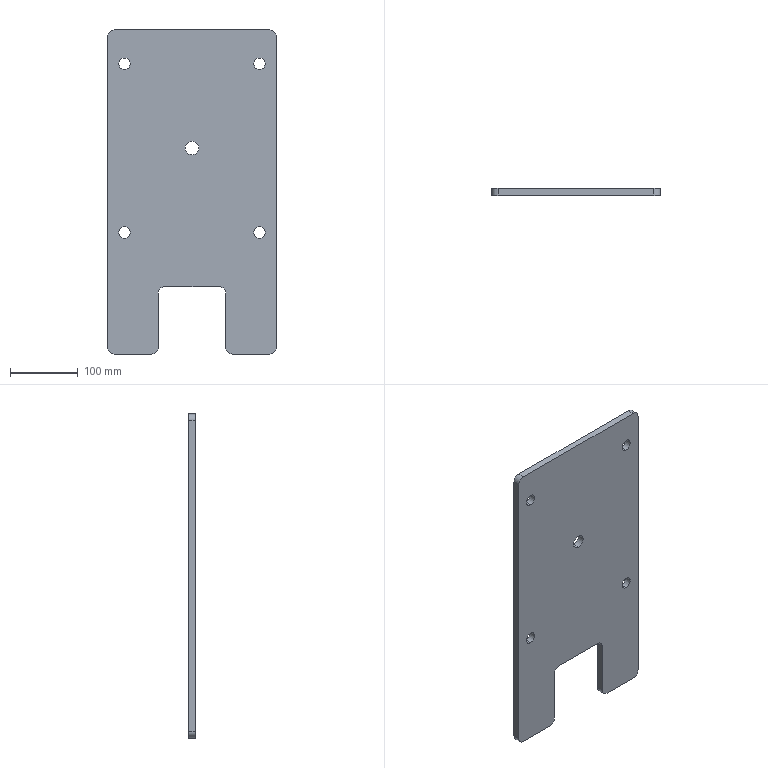Component | SolidWorks | Short-1_Finishing-1 | 1 solid | 28 faces | box 250 x 10 x 480 mm | volume 1086921 mm3 | cylinder 18 | plane 10 | commonest cylinder face diameters 20 x10 17 x8 | material Plain Carbon Steel
STEP:
#1=CARTESIAN_POINT('',(-127.449,-24.751,197.676));
#2=VERTEX_POINT('',#1);
#3=CARTESIAN_POINT('',(-127.449,-24.751,196.889));
#4=VERTEX_POINT('',#3);
#5=CARTESIAN_POINT('',(-127.449,-24.751,197.282));
#6=DIRECTION('',(0.,1.,-0.));
#7=DIRECTION('',(0.,0.,-1.));
#8=AXIS2_PLACEMENT_3D('',#5,#6,#7);
#9=CIRCLE('',#8,0.3937);
#10=EDGE_CURVE('',#2,#4,#9,.T.);
#11=ORIENTED_EDGE('',*,*,#10,.F.);
#12=CARTESIAN_POINT('',(-127.449,-24.357,197.676));
#13=VERTEX_POINT('',#12);
#14=CARTESIAN_POINT('',(-127.449,-24.751,197.676));
#15=DIRECTION('',(0.,1.,-0.));
#16=VECTOR('',#15,39.37);
#17=LINE('',#14,#16);
#18=EDGE_CURVE('',#2,#13,#17,.T.);
#19=ORIENTED_EDGE('',*,*,#18,.T.);
#20=CARTESIAN_POINT('',(-127.449,-24.357,196.889));
#21=VERTEX_POINT('',#20);
#22=CARTESIAN_POINT('',(-127.449,-24.357,197.282));
#23=DIRECTION('',(0.,1.,-0.));
#24=DIRECTION('',(0.,0.,-1.));
#25=AXIS2_PLACEMENT_3D('',#22,#23,#24);
#26=CIRCLE('',#25,0.3937);
#27=EDGE_CURVE('',#13,#21,#26,.T.);
#28=ORIENTED_EDGE('',*,*,#27,.T.);
#29=CARTESIAN_POINT('',(-127.449,-24.751,196.889));
#30=DIRECTION('',(0.,1.,-0.));
#31=VECTOR('',#30,39.37);
#32=LINE('',#29,#31);
#33=EDGE_CURVE('',#4,#21,#32,.T.);
#34=ORIENTED_EDGE('',*,*,#33,.F.);
#35=EDGE_LOOP('',(#11,#19,#28,#34));
#36=FACE_OUTER_BOUND('',#35,.T.);
#37=CARTESIAN_POINT('',(-127.449,-24.751,197.282));
#38=DIRECTION('',(0.,1.,-0.));
#39=DIRECTION('',(0.,0.,-1.));
#40=AXIS2_PLACEMENT_3D('',#37,#38,#39);
#41=CYLINDRICAL_SURFACE('',#40,0.3937);
#42=ADVANCED_FACE('',(#36),#41,.F.);
#43=CARTESIAN_POINT('',(-123.512,-24.751,202.538));
#44=VERTEX_POINT('',#43);
#45=CARTESIAN_POINT('',(-123.512,-24.751,201.869));
#46=VERTEX_POINT('',#45);
#47=CARTESIAN_POINT('',(-123.512,-24.751,202.204));
#48=DIRECTION('',(0.,1.,-0.));
#49=DIRECTION('',(0.,0.,1.));
#50=AXIS2_PLACEMENT_3D('',#47,#48,#49);
#51=CIRCLE('',#50,0.3346);
#52=EDGE_CURVE('',#44,#46,#51,.T.);
#53=ORIENTED_EDGE('',*,*,#52,.F.);
#54=CARTESIAN_POINT('',(-123.512,-24.357,202.538));
#55=VERTEX_POINT('',#54);
#56=CARTESIAN_POINT('',(-123.512,-24.751,202.538));
#57=DIRECTION('',(0.,1.,-0.));
#58=VECTOR('',#57,39.37);
#59=LINE('',#56,#58);
#60=EDGE_CURVE('',#44,#55,#59,.T.);
#61=ORIENTED_EDGE('',*,*,#60,.T.);
#62=CARTESIAN_POINT('',(-123.512,-24.357,201.869));
#63=VERTEX_POINT('',#62);
#64=CARTESIAN_POINT('',(-123.512,-24.357,202.204));
#65=DIRECTION('',(0.,1.,-0.));
#66=DIRECTION('',(0.,0.,1.));
#67=AXIS2_PLACEMENT_3D('',#64,#65,#66);
#68=CIRCLE('',#67,0.3346);
#69=EDGE_CURVE('',#55,#63,#68,.T.);
#70=ORIENTED_EDGE('',*,*,#69,.T.);
#71=CARTESIAN_POINT('',(-123.512,-24.751,201.869));
#72=DIRECTION('',(0.,1.,-0.));
#73=VECTOR('',#72,39.37);
#74=LINE('',#71,#73);
#75=EDGE_CURVE('',#46,#63,#74,.T.);
#76=ORIENTED_EDGE('',*,*,#75,.F.);
#77=EDGE_LOOP('',(#53,#61,#70,#76));
#78=FACE_OUTER_BOUND('',#77,.T.);
#79=CARTESIAN_POINT('',(-123.512,-24.751,202.204));
#80=DIRECTION('',(0.,1.,-0.));
#81=DIRECTION('',(0.,0.,-1.));
#82=AXIS2_PLACEMENT_3D('',#79,#80,#81);
#83=CYLINDRICAL_SURFACE('',#82,0.3346);
#84=ADVANCED_FACE('',(#78),#83,.F.);
#85=CARTESIAN_POINT('',(-123.512,-24.751,192.696));
#86=VERTEX_POINT('',#85);
#87=CARTESIAN_POINT('',(-123.512,-24.751,192.027));
#88=VERTEX_POINT('',#87);
#89=CARTESIAN_POINT('',(-123.512,-24.751,192.361));
#90=DIRECTION('',(0.,1.,-0.));
#91=DIRECTION('',(0.,0.,1.));
#92=AXIS2_PLACEMENT_3D('',#89,#90,#91);
#93=CIRCLE('',#92,0.3346);
#94=EDGE_CURVE('',#86,#88,#93,.T.);
#95=ORIENTED_EDGE('',*,*,#94,.F.);
#96=CARTESIAN_POINT('',(-123.512,-24.357,192.696));
#97=VERTEX_POINT('',#96);
#98=CARTESIAN_POINT('',(-123.512,-24.751,192.696));
#99=DIRECTION('',(0.,1.,-0.));
#100=VECTOR('',#99,39.37);
#101=LINE('',#98,#100);
#102=EDGE_CURVE('',#86,#97,#101,.T.);
#103=ORIENTED_EDGE('',*,*,#102,.T.);
#104=CARTESIAN_POINT('',(-123.512,-24.357,192.027));
#105=VERTEX_POINT('',#104);
#106=CARTESIAN_POINT('',(-123.512,-24.357,192.361));
#107=DIRECTION('',(0.,1.,-0.));
#108=DIRECTION('',(0.,0.,1.));
#109=AXIS2_PLACEMENT_3D('',#106,#107,#108);
#110=CIRCLE('',#109,0.3346);
#111=EDGE_CURVE('',#97,#105,#110,.T.);
#112=ORIENTED_EDGE('',*,*,#111,.T.);
#113=CARTESIAN_POINT('',(-123.512,-24.751,192.027));
#114=DIRECTION('',(0.,1.,-0.));
#115=VECTOR('',#114,39.37);
#116=LINE('',#113,#115);
#117=EDGE_CURVE('',#88,#105,#116,.T.);
#118=ORIENTED_EDGE('',*,*,#117,.F.);
#119=EDGE_LOOP('',(#95,#103,#112,#118));
#120=FACE_OUTER_BOUND('',#119,.T.);
#121=CARTESIAN_POINT('',(-123.512,-24.751,192.361));
#122=DIRECTION('',(0.,1.,-0.));
#123=DIRECTION('',(0.,0.,-1.));
#124=AXIS2_PLACEMENT_3D('',#121,#122,#123);
#125=CYLINDRICAL_SURFACE('',#124,0.3346);
#126=ADVANCED_FACE('',(#120),#125,.F.);
#127=CARTESIAN_POINT('',(-131.386,-24.751,192.696));
#128=VERTEX_POINT('',#127);
#129=CARTESIAN_POINT('',(-131.386,-24.751,192.027));
#130=VERTEX_POINT('',#129);
#131=CARTESIAN_POINT('',(-131.386,-24.751,192.361));
#132=DIRECTION('',(0.,1.,-0.));
#133=DIRECTION('',(0.,0.,-1.));
#134=AXIS2_PLACEMENT_3D('',#131,#132,#133);
#135=CIRCLE('',#134,0.3346);
#136=EDGE_CURVE('',#128,#130,#135,.T.);
#137=ORIENTED_EDGE('',*,*,#136,.F.);
#138=CARTESIAN_POINT('',(-131.386,-24.357,192.696));
#139=VERTEX_POINT('',#138);
#140=CARTESIAN_POINT('',(-131.386,-24.751,192.696));
#141=DIRECTION('',(0.,1.,-0.));
#142=VECTOR('',#141,39.37);
#143=LINE('',#140,#142);
#144=EDGE_CURVE('',#128,#139,#143,.T.);
#145=ORIENTED_EDGE('',*,*,#144,.T.);
#146=CARTESIAN_POINT('',(-131.386,-24.357,192.027));
#147=VERTEX_POINT('',#146);
#148=CARTESIAN_POINT('',(-131.386,-24.357,192.361));
#149=DIRECTION('',(0.,1.,-0.));
#150=DIRECTION('',(0.,0.,-1.));
#151=AXIS2_PLACEMENT_3D('',#148,#149,#150);
#152=CIRCLE('',#151,0.3346);
#153=EDGE_CURVE('',#139,#147,#152,.T.);
#154=ORIENTED_EDGE('',*,*,#153,.T.);
#155=CARTESIAN_POINT('',(-131.386,-24.751,192.027));
#156=DIRECTION('',(0.,1.,-0.));
#157=VECTOR('',#156,39.37);
#158=LINE('',#155,#157);
#159=EDGE_CURVE('',#130,#147,#158,.T.);
#160=ORIENTED_EDGE('',*,*,#159,.F.);
#161=EDGE_LOOP('',(#137,#145,#154,#160));
#162=FACE_OUTER_BOUND('',#161,.T.);
#163=CARTESIAN_POINT('',(-131.386,-24.751,192.361));
#164=DIRECTION('',(0.,1.,-0.));
#165=DIRECTION('',(0.,0.,-1.));
#166=AXIS2_PLACEMENT_3D('',#163,#164,#165);
#167=CYLINDRICAL_SURFACE('',#166,0.3346);
#168=ADVANCED_FACE('',(#162),#167,.F.);
#169=CARTESIAN_POINT('',(-131.386,-24.751,202.538));
#170=VERTEX_POINT('',#169);
#171=CARTESIAN_POINT('',(-131.386,-24.751,201.869));
#172=VERTEX_POINT('',#171);
#173=CARTESIAN_POINT('',(-131.386,-24.751,202.204));
#174=DIRECTION('',(0.,1.,-0.));
#175=DIRECTION('',(0.,0.,-1.));
#176=AXIS2_PLACEMENT_3D('',#173,#174,#175);
#177=CIRCLE('',#176,0.3346);
#178=EDGE_CURVE('',#170,#172,#177,.T.);
#179=ORIENTED_EDGE('',*,*,#178,.F.);
#180=CARTESIAN_POINT('',(-131.386,-24.357,202.538));
#181=VERTEX_POINT('',#180);
#182=CARTESIAN_POINT('',(-131.386,-24.751,202.538));
#183=DIRECTION('',(0.,1.,-0.));
#184=VECTOR('',#183,39.37);
#185=LINE('',#182,#184);
#186=EDGE_CURVE('',#170,#181,#185,.T.);
#187=ORIENTED_EDGE('',*,*,#186,.T.);
#188=CARTESIAN_POINT('',(-131.386,-24.357,201.869));
#189=VERTEX_POINT('',#188);
#190=CARTESIAN_POINT('',(-131.386,-24.357,202.204));
#191=DIRECTION('',(0.,1.,-0.));
#192=DIRECTION('',(0.,0.,-1.));
#193=AXIS2_PLACEMENT_3D('',#190,#191,#192);
#194=CIRCLE('',#193,0.3346);
#195=EDGE_CURVE('',#181,#189,#194,.T.);
#196=ORIENTED_EDGE('',*,*,#195,.T.);
#197=CARTESIAN_POINT('',(-131.386,-24.751,201.869));
#198=DIRECTION('',(0.,1.,-0.));
#199=VECTOR('',#198,39.37);
#200=LINE('',#197,#199);
#201=EDGE_CURVE('',#172,#189,#200,.T.);
#202=ORIENTED_EDGE('',*,*,#201,.F.);
#203=EDGE_LOOP('',(#179,#187,#196,#202));
#204=FACE_OUTER_BOUND('',#203,.T.);
#205=CARTESIAN_POINT('',(-131.386,-24.751,202.204));
#206=DIRECTION('',(0.,1.,-0.));
#207=DIRECTION('',(0.,0.,-1.));
#208=AXIS2_PLACEMENT_3D('',#205,#206,#207);
#209=CYLINDRICAL_SURFACE('',#208,0.3346);
#210=ADVANCED_FACE('',(#204),#209,.F.);
#211=CARTESIAN_POINT('',(-125.48,-24.357,188.818));
#212=VERTEX_POINT('',#211);
#213=CARTESIAN_POINT('',(-125.874,-24.357,189.212));
#214=VERTEX_POINT('',#213);
#215=CARTESIAN_POINT('',(-125.874,-24.357,188.818));
#216=DIRECTION('',(-0.,-1.,0.));
#217=DIRECTION('',(0.,0.,-1.));
#218=AXIS2_PLACEMENT_3D('',#215,#216,#217);
#219=CIRCLE('',#218,0.3937);
#220=EDGE_CURVE('',#212,#214,#219,.T.);
#221=ORIENTED_EDGE('',*,*,#220,.F.);
#222=CARTESIAN_POINT('',(-125.48,-24.751,188.818));
#223=VERTEX_POINT('',#222);
#224=CARTESIAN_POINT('',(-125.48,-24.751,188.818));
#225=DIRECTION('',(0.,1.,-0.));
#226=VECTOR('',#225,39.37);
#227=LINE('',#224,#226);
#228=EDGE_CURVE('',#223,#212,#227,.T.);
#229=ORIENTED_EDGE('',*,*,#228,.F.);
#230=CARTESIAN_POINT('',(-125.874,-24.751,189.212));
#231=VERTEX_POINT('',#230);
#232=CARTESIAN_POINT('',(-125.874,-24.751,188.818));
#233=DIRECTION('',(-0.,-1.,0.));
#234=DIRECTION('',(0.,0.,-1.));
#235=AXIS2_PLACEMENT_3D('',#232,#233,#234);
#236=CIRCLE('',#235,0.3937);
#237=EDGE_CURVE('',#223,#231,#236,.T.);
#238=ORIENTED_EDGE('',*,*,#237,.T.);
#239=CARTESIAN_POINT('',(-125.874,-24.751,189.212));
#240=DIRECTION('',(0.,1.,-0.));
#241=VECTOR('',#240,39.37);
#242=LINE('',#239,#241);
#243=EDGE_CURVE('',#231,#214,#242,.T.);
#244=ORIENTED_EDGE('',*,*,#243,.T.);
#245=EDGE_LOOP('',(#221,#229,#238,#244));
#246=FACE_OUTER_BOUND('',#245,.T.);
#247=CARTESIAN_POINT('',(-125.874,-24.751,188.818));
#248=DIRECTION('',(0.,1.,-0.));
#249=DIRECTION('',(0.,0.,-1.));
#250=AXIS2_PLACEMENT_3D('',#247,#248,#249);
#251=CYLINDRICAL_SURFACE('',#250,0.3937);
#252=ADVANCED_FACE('',(#246),#251,.F.);
#253=CARTESIAN_POINT('',(-125.48,-24.357,185.668));
#254=VERTEX_POINT('',#253);
#255=CARTESIAN_POINT('',(-125.48,-24.357,188.818));
#256=DIRECTION('',(0.,0.,1.));
#257=VECTOR('',#256,39.37);
#258=LINE('',#255,#257);
#259=EDGE_CURVE('',#254,#212,#258,.T.);
#260=ORIENTED_EDGE('',*,*,#259,.F.);
#261=CARTESIAN_POINT('',(-125.48,-24.751,185.668));
#262=VERTEX_POINT('',#261);
#263=CARTESIAN_POINT('',(-125.48,-24.751,185.668));
#264=DIRECTION('',(0.,1.,-0.));
#265=VECTOR('',#264,39.37);
#266=LINE('',#263,#265);
#267=EDGE_CURVE('',#262,#254,#266,.T.);
#268=ORIENTED_EDGE('',*,*,#267,.F.);
#269=CARTESIAN_POINT('',(-125.48,-24.751,188.818));
#270=DIRECTION('',(0.,0.,1.));
#271=VECTOR('',#270,39.37);
#272=LINE('',#269,#271);
#273=EDGE_CURVE('',#262,#223,#272,.T.);
#274=ORIENTED_EDGE('',*,*,#273,.T.);
#275=ORIENTED_EDGE('',*,*,#228,.T.);
#276=EDGE_LOOP('',(#260,#268,#274,#275));
#277=FACE_OUTER_BOUND('',#276,.T.);
#278=CARTESIAN_POINT('',(-125.48,-24.751,188.818));
#279=DIRECTION('',(-1.,0.,0.));
#280=DIRECTION('',(0.,0.,1.));
#281=AXIS2_PLACEMENT_3D('',#278,#279,#280);
#282=PLANE('',#281);
#283=ADVANCED_FACE('',(#277),#282,.T.);
#284=CARTESIAN_POINT('',(-125.087,-24.357,185.275));
#285=VERTEX_POINT('',#284);
#286=CARTESIAN_POINT('',(-125.087,-24.357,185.668));
#287=DIRECTION('',(0.,1.,-0.));
#288=DIRECTION('',(0.,0.,1.));
#289=AXIS2_PLACEMENT_3D('',#286,#287,#288);
#290=CIRCLE('',#289,0.3937);
#291=EDGE_CURVE('',#285,#254,#290,.T.);
#292=ORIENTED_EDGE('',*,*,#291,.F.);
#293=CARTESIAN_POINT('',(-125.087,-24.751,185.275));
#294=VERTEX_POINT('',#293);
#295=CARTESIAN_POINT('',(-125.087,-24.751,185.275));
#296=DIRECTION('',(0.,1.,-0.));
#297=VECTOR('',#296,39.37);
#298=LINE('',#295,#297);
#299=EDGE_CURVE('',#294,#285,#298,.T.);
#300=ORIENTED_EDGE('',*,*,#299,.F.);
#301=CARTESIAN_POINT('',(-125.087,-24.751,185.668));
#302=DIRECTION('',(0.,1.,-0.));
#303=DIRECTION('',(0.,0.,1.));
#304=AXIS2_PLACEMENT_3D('',#301,#302,#303);
#305=CIRCLE('',#304,0.3937);
#306=EDGE_CURVE('',#294,#262,#305,.T.);
#307=ORIENTED_EDGE('',*,*,#306,.T.);
#308=ORIENTED_EDGE('',*,*,#267,.T.);
#309=EDGE_LOOP('',(#292,#300,#307,#308));
#310=FACE_OUTER_BOUND('',#309,.T.);
#311=CARTESIAN_POINT('',(-125.087,-24.751,185.668));
#312=DIRECTION('',(0.,1.,-0.));
#313=DIRECTION('',(0.,0.,-1.));
#314=AXIS2_PLACEMENT_3D('',#311,#312,#313);
#315=CYLINDRICAL_SURFACE('',#314,0.3937);
#316=ADVANCED_FACE('',(#310),#315,.T.);
#317=CARTESIAN_POINT('',(-122.921,-24.357,185.275));
#318=VERTEX_POINT('',#317);
#319=CARTESIAN_POINT('',(-125.087,-24.357,185.275));
#320=DIRECTION('',(-1.,0.,0.));
#321=VECTOR('',#320,39.37);
#322=LINE('',#319,#321);
#323=EDGE_CURVE('',#318,#285,#322,.T.);
#324=ORIENTED_EDGE('',*,*,#323,.F.);
#325=CARTESIAN_POINT('',(-122.921,-24.751,185.275));
#326=VERTEX_POINT('',#325);
#327=CARTESIAN_POINT('',(-122.921,-24.751,185.275));
#328=DIRECTION('',(0.,1.,-0.));
#329=VECTOR('',#328,39.37);
#330=LINE('',#327,#329);
#331=EDGE_CURVE('',#326,#318,#330,.T.);
#332=ORIENTED_EDGE('',*,*,#331,.F.);
#333=CARTESIAN_POINT('',(-125.087,-24.751,185.275));
#334=DIRECTION('',(-1.,0.,0.));
#335=VECTOR('',#334,39.37);
#336=LINE('',#333,#335);
#337=EDGE_CURVE('',#326,#294,#336,.T.);
#338=ORIENTED_EDGE('',*,*,#337,.T.);
#339=ORIENTED_EDGE('',*,*,#299,.T.);
#340=EDGE_LOOP('',(#324,#332,#338,#339));
#341=FACE_OUTER_BOUND('',#340,.T.);
#342=CARTESIAN_POINT('',(-125.087,-24.751,185.275));
#343=DIRECTION('',(-0.,-0.,-1.));
#344=DIRECTION('',(-1.,0.,0.));
#345=AXIS2_PLACEMENT_3D('',#342,#343,#344);
#346=PLANE('',#345);
#347=ADVANCED_FACE('',(#341),#346,.T.);
#348=CARTESIAN_POINT('',(-122.528,-24.357,185.668));
#349=VERTEX_POINT('',#348);
#350=CARTESIAN_POINT('',(-122.921,-24.357,185.668));
#351=DIRECTION('',(0.,1.,-0.));
#352=DIRECTION('',(0.,0.,1.));
#353=AXIS2_PLACEMENT_3D('',#350,#351,#352);
#354=CIRCLE('',#353,0.3937);
#355=EDGE_CURVE('',#349,#318,#354,.T.);
#356=ORIENTED_EDGE('',*,*,#355,.F.);
#357=CARTESIAN_POINT('',(-122.528,-24.751,185.668));
#358=VERTEX_POINT('',#357);
#359=CARTESIAN_POINT('',(-122.528,-24.751,185.668));
#360=DIRECTION('',(0.,1.,-0.));
#361=VECTOR('',#360,39.37);
#362=LINE('',#359,#361);
#363=EDGE_CURVE('',#358,#349,#362,.T.);
#364=ORIENTED_EDGE('',*,*,#363,.F.);
#365=CARTESIAN_POINT('',(-122.921,-24.751,185.668));
#366=DIRECTION('',(0.,1.,-0.));
#367=DIRECTION('',(0.,0.,1.));
#368=AXIS2_PLACEMENT_3D('',#365,#366,#367);
#369=CIRCLE('',#368,0.3937);
#370=EDGE_CURVE('',#358,#326,#369,.T.);
#371=ORIENTED_EDGE('',*,*,#370,.T.);
#372=ORIENTED_EDGE('',*,*,#331,.T.);
#373=EDGE_LOOP('',(#356,#364,#371,#372));
#374=FACE_OUTER_BOUND('',#373,.T.);
#375=CARTESIAN_POINT('',(-122.921,-24.751,185.668));
#376=DIRECTION('',(0.,1.,-0.));
#377=DIRECTION('',(0.,0.,-1.));
#378=AXIS2_PLACEMENT_3D('',#375,#376,#377);
#379=CYLINDRICAL_SURFACE('',#378,0.3937);
#380=ADVANCED_FACE('',(#374),#379,.T.);
#381=CARTESIAN_POINT('',(-122.528,-24.357,203.778));
#382=VERTEX_POINT('',#381);
#383=CARTESIAN_POINT('',(-122.528,-24.357,185.668));
#384=DIRECTION('',(-0.,-0.,-1.));
#385=VECTOR('',#384,39.37);
#386=LINE('',#383,#385);
#387=EDGE_CURVE('',#382,#349,#386,.T.);
#388=ORIENTED_EDGE('',*,*,#387,.F.);
#389=CARTESIAN_POINT('',(-122.528,-24.751,203.778));
#390=VERTEX_POINT('',#389);
#391=CARTESIAN_POINT('',(-122.528,-24.751,203.778));
#392=DIRECTION('',(0.,1.,-0.));
#393=VECTOR('',#392,39.37);
#394=LINE('',#391,#393);
#395=EDGE_CURVE('',#390,#382,#394,.T.);
#396=ORIENTED_EDGE('',*,*,#395,.F.);
#397=CARTESIAN_POINT('',(-122.528,-24.751,185.668));
#398=DIRECTION('',(-0.,-0.,-1.));
#399=VECTOR('',#398,39.37);
#400=LINE('',#397,#399);
#401=EDGE_CURVE('',#390,#358,#400,.T.);
#402=ORIENTED_EDGE('',*,*,#401,.T.);
#403=ORIENTED_EDGE('',*,*,#363,.T.);
#404=EDGE_LOOP('',(#388,#396,#402,#403));
#405=FACE_OUTER_BOUND('',#404,.T.);
#406=CARTESIAN_POINT('',(-122.528,-24.751,185.668));
#407=DIRECTION('',(1.,-0.,0.));
#408=DIRECTION('',(-0.,-0.,-1.));
#409=AXIS2_PLACEMENT_3D('',#406,#407,#408);
#410=PLANE('',#409);
#411=ADVANCED_FACE('',(#405),#410,.T.);
#412=CARTESIAN_POINT('',(-122.921,-24.357,204.172));
#413=VERTEX_POINT('',#412);
#414=CARTESIAN_POINT('',(-122.921,-24.357,203.778));
#415=DIRECTION('',(0.,1.,-0.));
#416=DIRECTION('',(0.,0.,-1.));
#417=AXIS2_PLACEMENT_3D('',#414,#415,#416);
#418=CIRCLE('',#417,0.3937);
#419=EDGE_CURVE('',#413,#382,#418,.T.);
#420=ORIENTED_EDGE('',*,*,#419,.F.);
#421=CARTESIAN_POINT('',(-122.921,-24.751,204.172));
#422=VERTEX_POINT('',#421);
#423=CARTESIAN_POINT('',(-122.921,-24.751,204.172));
#424=DIRECTION('',(0.,1.,-0.));
#425=VECTOR('',#424,39.37);
#426=LINE('',#423,#425);
#427=EDGE_CURVE('',#422,#413,#426,.T.);
#428=ORIENTED_EDGE('',*,*,#427,.F.);
#429=CARTESIAN_POINT('',(-122.921,-24.751,203.778));
#430=DIRECTION('',(0.,1.,-0.));
#431=DIRECTION('',(0.,0.,-1.));
#432=AXIS2_PLACEMENT_3D('',#429,#430,#431);
#433=CIRCLE('',#432,0.3937);
#434=EDGE_CURVE('',#422,#390,#433,.T.);
#435=ORIENTED_EDGE('',*,*,#434,.T.);
#436=ORIENTED_EDGE('',*,*,#395,.T.);
#437=EDGE_LOOP('',(#420,#428,#435,#436));
#438=FACE_OUTER_BOUND('',#437,.T.);
#439=CARTESIAN_POINT('',(-122.921,-24.751,203.778));
#440=DIRECTION('',(0.,1.,-0.));
#441=DIRECTION('',(0.,0.,-1.));
#442=AXIS2_PLACEMENT_3D('',#439,#440,#441);
#443=CYLINDRICAL_SURFACE('',#442,0.3937);
#444=ADVANCED_FACE('',(#438),#443,.T.);
#445=CARTESIAN_POINT('',(-131.976,-24.357,204.172));
#446=VERTEX_POINT('',#445);
#447=CARTESIAN_POINT('',(-122.921,-24.357,204.172));
#448=DIRECTION('',(1.,-0.,0.));
#449=VECTOR('',#448,39.37);
#450=LINE('',#447,#449);
#451=EDGE_CURVE('',#446,#413,#450,.T.);
#452=ORIENTED_EDGE('',*,*,#451,.F.);
#453=CARTESIAN_POINT('',(-131.976,-24.751,204.172));
#454=VERTEX_POINT('',#453);
#455=CARTESIAN_POINT('',(-131.976,-24.751,204.172));
#456=DIRECTION('',(0.,1.,-0.));
#457=VECTOR('',#456,39.37);
#458=LINE('',#455,#457);
#459=EDGE_CURVE('',#454,#446,#458,.T.);
#460=ORIENTED_EDGE('',*,*,#459,.F.);
#461=CARTESIAN_POINT('',(-122.921,-24.751,204.172));
#462=DIRECTION('',(1.,-0.,0.));
#463=VECTOR('',#462,39.37);
#464=LINE('',#461,#463);
#465=EDGE_CURVE('',#454,#422,#464,.T.);
#466=ORIENTED_EDGE('',*,*,#465,.T.);
#467=ORIENTED_EDGE('',*,*,#427,.T.);
#468=EDGE_LOOP('',(#452,#460,#466,#467));
#469=FACE_OUTER_BOUND('',#468,.T.);
#470=CARTESIAN_POINT('',(-122.921,-24.751,204.172));
#471=DIRECTION('',(0.,0.,1.));
#472=DIRECTION('',(1.,-0.,0.));
#473=AXIS2_PLACEMENT_3D('',#470,#471,#472);
#474=PLANE('',#473);
#475=ADVANCED_FACE('',(#469),#474,.T.);
#476=CARTESIAN_POINT('',(-132.37,-24.357,203.778));
#477=VERTEX_POINT('',#476);
#478=CARTESIAN_POINT('',(-131.976,-24.357,203.778));
#479=DIRECTION('',(0.,1.,-0.));
#480=DIRECTION('',(0.,0.,1.));
#481=AXIS2_PLACEMENT_3D('',#478,#479,#480);
#482=CIRCLE('',#481,0.3937);
#483=EDGE_CURVE('',#477,#446,#482,.T.);
#484=ORIENTED_EDGE('',*,*,#483,.F.);
#485=CARTESIAN_POINT('',(-132.37,-24.751,203.778));
#486=VERTEX_POINT('',#485);
#487=CARTESIAN_POINT('',(-132.37,-24.751,203.778));
#488=DIRECTION('',(0.,1.,-0.));
#489=VECTOR('',#488,39.37);
#490=LINE('',#487,#489);
#491=EDGE_CURVE('',#486,#477,#490,.T.);
#492=ORIENTED_EDGE('',*,*,#491,.F.);
#493=CARTESIAN_POINT('',(-131.976,-24.751,203.778));
#494=DIRECTION('',(0.,1.,-0.));
#495=DIRECTION('',(0.,0.,1.));
#496=AXIS2_PLACEMENT_3D('',#493,#494,#495);
#497=CIRCLE('',#496,0.3937);
#498=EDGE_CURVE('',#486,#454,#497,.T.);
#499=ORIENTED_EDGE('',*,*,#498,.T.);
#500=ORIENTED_EDGE('',*,*,#459,.T.);
#501=EDGE_LOOP('',(#484,#492,#499,#500));
#502=FACE_OUTER_BOUND('',#501,.T.);
#503=CARTESIAN_POINT('',(-131.976,-24.751,203.778));
#504=DIRECTION('',(0.,1.,-0.));
#505=DIRECTION('',(0.,0.,-1.));
#506=AXIS2_PLACEMENT_3D('',#503,#504,#505);
#507=CYLINDRICAL_SURFACE('',#506,0.3937);
#508=ADVANCED_FACE('',(#502),#507,.T.);
#509=CARTESIAN_POINT('',(-132.37,-24.357,185.668));
#510=VERTEX_POINT('',#509);
#511=CARTESIAN_POINT('',(-132.37,-24.357,203.778));
#512=DIRECTION('',(0.,0.,1.));
#513=VECTOR('',#512,39.37);
#514=LINE('',#511,#513);
#515=EDGE_CURVE('',#510,#477,#514,.T.);
#516=ORIENTED_EDGE('',*,*,#515,.F.);
#517=CARTESIAN_POINT('',(-132.37,-24.751,185.668));
#518=VERTEX_POINT('',#517);
#519=CARTESIAN_POINT('',(-132.37,-24.751,185.668));
#520=DIRECTION('',(0.,1.,-0.));
#521=VECTOR('',#520,39.37);
#522=LINE('',#519,#521);
#523=EDGE_CURVE('',#518,#510,#522,.T.);
#524=ORIENTED_EDGE('',*,*,#523,.F.);
#525=CARTESIAN_POINT('',(-132.37,-24.751,203.778));
#526=DIRECTION('',(0.,0.,1.));
#527=VECTOR('',#526,39.37);
#528=LINE('',#525,#527);
#529=EDGE_CURVE('',#518,#486,#528,.T.);
#530=ORIENTED_EDGE('',*,*,#529,.T.);
#531=ORIENTED_EDGE('',*,*,#491,.T.);
#532=EDGE_LOOP('',(#516,#524,#530,#531));
#533=FACE_OUTER_BOUND('',#532,.T.);
#534=CARTESIAN_POINT('',(-132.37,-24.751,203.778));
#535=DIRECTION('',(-1.,0.,0.));
#536=DIRECTION('',(0.,0.,1.));
#537=AXIS2_PLACEMENT_3D('',#534,#535,#536);
#538=PLANE('',#537);
#539=ADVANCED_FACE('',(#533),#538,.T.);
#540=CARTESIAN_POINT('',(-131.976,-24.357,185.275));
#541=VERTEX_POINT('',#540);
#542=CARTESIAN_POINT('',(-131.976,-24.357,185.668));
#543=DIRECTION('',(0.,1.,-0.));
#544=DIRECTION('',(0.,0.,1.));
#545=AXIS2_PLACEMENT_3D('',#542,#543,#544);
#546=CIRCLE('',#545,0.3937);
#547=EDGE_CURVE('',#541,#510,#546,.T.);
#548=ORIENTED_EDGE('',*,*,#547,.F.);
#549=CARTESIAN_POINT('',(-131.976,-24.751,185.275));
#550=VERTEX_POINT('',#549);
#551=CARTESIAN_POINT('',(-131.976,-24.751,185.275));
#552=DIRECTION('',(0.,1.,-0.));
#553=VECTOR('',#552,39.37);
#554=LINE('',#551,#553);
#555=EDGE_CURVE('',#550,#541,#554,.T.);
#556=ORIENTED_EDGE('',*,*,#555,.F.);
#557=CARTESIAN_POINT('',(-131.976,-24.751,185.668));
#558=DIRECTION('',(0.,1.,-0.));
#559=DIRECTION('',(0.,0.,1.));
#560=AXIS2_PLACEMENT_3D('',#557,#558,#559);
#561=CIRCLE('',#560,0.3937);
#562=EDGE_CURVE('',#550,#518,#561,.T.);
#563=ORIENTED_EDGE('',*,*,#562,.T.);
#564=ORIENTED_EDGE('',*,*,#523,.T.);
#565=EDGE_LOOP('',(#548,#556,#563,#564));
#566=FACE_OUTER_BOUND('',#565,.T.);
#567=CARTESIAN_POINT('',(-131.976,-24.751,185.668));
#568=DIRECTION('',(0.,1.,-0.));
#569=DIRECTION('',(0.,0.,-1.));
#570=AXIS2_PLACEMENT_3D('',#567,#568,#569);
#571=CYLINDRICAL_SURFACE('',#570,0.3937);
#572=ADVANCED_FACE('',(#566),#571,.T.);
#573=CARTESIAN_POINT('',(-129.811,-24.357,185.275));
#574=VERTEX_POINT('',#573);
#575=CARTESIAN_POINT('',(-131.976,-24.357,185.275));
#576=DIRECTION('',(-1.,0.,0.));
#577=VECTOR('',#576,39.37);
#578=LINE('',#575,#577);
#579=EDGE_CURVE('',#574,#541,#578,.T.);
#580=ORIENTED_EDGE('',*,*,#579,.F.);
#581=CARTESIAN_POINT('',(-129.811,-24.751,185.275));
#582=VERTEX_POINT('',#581);
#583=CARTESIAN_POINT('',(-129.811,-24.751,185.275));
#584=DIRECTION('',(0.,1.,-0.));
#585=VECTOR('',#584,39.37);
#586=LINE('',#583,#585);
#587=EDGE_CURVE('',#582,#574,#586,.T.);
#588=ORIENTED_EDGE('',*,*,#587,.F.);
#589=CARTESIAN_POINT('',(-131.976,-24.751,185.275));
#590=DIRECTION('',(-1.,0.,0.));
#591=VECTOR('',#590,39.37);
#592=LINE('',#589,#591);
#593=EDGE_CURVE('',#582,#550,#592,.T.);
#594=ORIENTED_EDGE('',*,*,#593,.T.);
#595=ORIENTED_EDGE('',*,*,#555,.T.);
#596=EDGE_LOOP('',(#580,#588,#594,#595));
#597=FACE_OUTER_BOUND('',#596,.T.);
#598=CARTESIAN_POINT('',(-131.976,-24.751,185.275));
#599=DIRECTION('',(-0.,-0.,-1.));
#600=DIRECTION('',(-1.,0.,0.));
#601=AXIS2_PLACEMENT_3D('',#598,#599,#600);
#602=PLANE('',#601);
#603=ADVANCED_FACE('',(#597),#602,.T.);
#604=CARTESIAN_POINT('',(-129.417,-24.357,185.668));
#605=VERTEX_POINT('',#604);
#606=CARTESIAN_POINT('',(-129.811,-24.357,185.668));
#607=DIRECTION('',(0.,1.,-0.));
#608=DIRECTION('',(0.,0.,1.));
#609=AXIS2_PLACEMENT_3D('',#606,#607,#608);
#610=CIRCLE('',#609,0.3937);
#611=EDGE_CURVE('',#605,#574,#610,.T.);
#612=ORIENTED_EDGE('',*,*,#611,.F.);
#613=CARTESIAN_POINT('',(-129.417,-24.751,185.668));
#614=VERTEX_POINT('',#613);
#615=CARTESIAN_POINT('',(-129.417,-24.751,185.668));
#616=DIRECTION('',(0.,1.,-0.));
#617=VECTOR('',#616,39.37);
#618=LINE('',#615,#617);
#619=EDGE_CURVE('',#614,#605,#618,.T.);
#620=ORIENTED_EDGE('',*,*,#619,.F.);
#621=CARTESIAN_POINT('',(-129.811,-24.751,185.668));
#622=DIRECTION('',(0.,1.,-0.));
#623=DIRECTION('',(0.,0.,1.));
#624=AXIS2_PLACEMENT_3D('',#621,#622,#623);
#625=CIRCLE('',#624,0.3937);
#626=EDGE_CURVE('',#614,#582,#625,.T.);
#627=ORIENTED_EDGE('',*,*,#626,.T.);
#628=ORIENTED_EDGE('',*,*,#587,.T.);
#629=EDGE_LOOP('',(#612,#620,#627,#628));
#630=FACE_OUTER_BOUND('',#629,.T.);
#631=CARTESIAN_POINT('',(-129.811,-24.751,185.668));
#632=DIRECTION('',(0.,1.,-0.));
#633=DIRECTION('',(0.,0.,-1.));
#634=AXIS2_PLACEMENT_3D('',#631,#632,#633);
#635=CYLINDRICAL_SURFACE('',#634,0.3937);
#636=ADVANCED_FACE('',(#630),#635,.T.);
#637=CARTESIAN_POINT('',(-129.417,-24.357,188.818));
#638=VERTEX_POINT('',#637);
#639=CARTESIAN_POINT('',(-129.417,-24.357,185.668));
#640=DIRECTION('',(-0.,-0.,-1.));
#641=VECTOR('',#640,39.37);
#642=LINE('',#639,#641);
#643=EDGE_CURVE('',#638,#605,#642,.T.);
#644=ORIENTED_EDGE('',*,*,#643,.F.);
#645=CARTESIAN_POINT('',(-129.417,-24.751,188.818));
#646=VERTEX_POINT('',#645);
#647=CARTESIAN_POINT('',(-129.417,-24.751,188.818));
#648=DIRECTION('',(0.,1.,-0.));
#649=VECTOR('',#648,39.37);
#650=LINE('',#647,#649);
#651=EDGE_CURVE('',#646,#638,#650,.T.);
#652=ORIENTED_EDGE('',*,*,#651,.F.);
#653=CARTESIAN_POINT('',(-129.417,-24.751,185.668));
#654=DIRECTION('',(-0.,-0.,-1.));
#655=VECTOR('',#654,39.37);
#656=LINE('',#653,#655);
#657=EDGE_CURVE('',#646,#614,#656,.T.);
#658=ORIENTED_EDGE('',*,*,#657,.T.);
#659=ORIENTED_EDGE('',*,*,#619,.T.);
#660=EDGE_LOOP('',(#644,#652,#658,#659));
#661=FACE_OUTER_BOUND('',#660,.T.);
#662=CARTESIAN_POINT('',(-129.417,-24.751,185.668));
#663=DIRECTION('',(1.,-0.,0.));
#664=DIRECTION('',(-0.,-0.,-1.));
#665=AXIS2_PLACEMENT_3D('',#662,#663,#664);
#666=PLANE('',#665);
#667=ADVANCED_FACE('',(#661),#666,.T.);
#668=CARTESIAN_POINT('',(-129.024,-24.357,189.212));
#669=VERTEX_POINT('',#668);
#670=CARTESIAN_POINT('',(-129.024,-24.357,188.818));
#671=DIRECTION('',(-0.,-1.,0.));
#672=DIRECTION('',(0.,0.,-1.));
#673=AXIS2_PLACEMENT_3D('',#670,#671,#672);
#674=CIRCLE('',#673,0.3937);
#675=EDGE_CURVE('',#669,#638,#674,.T.);
#676=ORIENTED_EDGE('',*,*,#675,.F.);
#677=CARTESIAN_POINT('',(-129.024,-24.751,189.212));
#678=VERTEX_POINT('',#677);
#679=CARTESIAN_POINT('',(-129.024,-24.751,189.212));
#680=DIRECTION('',(0.,1.,-0.));
#681=VECTOR('',#680,39.37);
#682=LINE('',#679,#681);
#683=EDGE_CURVE('',#678,#669,#682,.T.);
#684=ORIENTED_EDGE('',*,*,#683,.F.);
#685=CARTESIAN_POINT('',(-129.024,-24.751,188.818));
#686=DIRECTION('',(-0.,-1.,0.));
#687=DIRECTION('',(0.,0.,-1.));
#688=AXIS2_PLACEMENT_3D('',#685,#686,#687);
#689=CIRCLE('',#688,0.3937);
#690=EDGE_CURVE('',#678,#646,#689,.T.);
#691=ORIENTED_EDGE('',*,*,#690,.T.);
#692=ORIENTED_EDGE('',*,*,#651,.T.);
#693=EDGE_LOOP('',(#676,#684,#691,#692));
#694=FACE_OUTER_BOUND('',#693,.T.);
#695=CARTESIAN_POINT('',(-129.024,-24.751,188.818));
#696=DIRECTION('',(0.,1.,-0.));
#697=DIRECTION('',(0.,0.,-1.));
#698=AXIS2_PLACEMENT_3D('',#695,#696,#697);
#699=CYLINDRICAL_SURFACE('',#698,0.3937);
#700=ADVANCED_FACE('',(#694),#699,.F.);
#701=CARTESIAN_POINT('',(-129.024,-24.357,189.212));
#702=DIRECTION('',(-1.,0.,-0.));
#703=VECTOR('',#702,39.37);
#704=LINE('',#701,#703);
#705=EDGE_CURVE('',#214,#669,#704,.T.);
#706=ORIENTED_EDGE('',*,*,#705,.F.);
#707=ORIENTED_EDGE('',*,*,#243,.F.);
#708=CARTESIAN_POINT('',(-129.024,-24.751,189.212));
#709=DIRECTION('',(-1.,0.,-0.));
#710=VECTOR('',#709,39.37);
#711=LINE('',#708,#710);
#712=EDGE_CURVE('',#231,#678,#711,.T.);
#713=ORIENTED_EDGE('',*,*,#712,.T.);
#714=ORIENTED_EDGE('',*,*,#683,.T.);
#715=EDGE_LOOP('',(#706,#707,#713,#714));
#716=FACE_OUTER_BOUND('',#715,.T.);
#717=CARTESIAN_POINT('',(-129.024,-24.751,189.212));
#718=DIRECTION('',(-0.,-0.,-1.));
#719=DIRECTION('',(-1.,0.,-0.));
#720=AXIS2_PLACEMENT_3D('',#717,#718,#719);
#721=PLANE('',#720);
#722=ADVANCED_FACE('',(#716),#721,.T.);
#723=CARTESIAN_POINT('',(-127.449,-24.751,197.282));
#724=DIRECTION('',(0.,1.,-0.));
#725=DIRECTION('',(0.,0.,-1.));
#726=AXIS2_PLACEMENT_3D('',#723,#724,#725);
#727=CIRCLE('',#726,0.3937);
#728=EDGE_CURVE('',#4,#2,#727,.T.);
#729=ORIENTED_EDGE('',*,*,#728,.T.);
#730=ORIENTED_EDGE('',*,*,#10,.T.);
#731=EDGE_LOOP('',(#729,#730));
#732=FACE_BOUND('',#731,.T.);
#733=CARTESIAN_POINT('',(-123.512,-24.751,202.204));
#734=DIRECTION('',(0.,1.,-0.));
#735=DIRECTION('',(0.,0.,1.));
#736=AXIS2_PLACEMENT_3D('',#733,#734,#735);
#737=CIRCLE('',#736,0.3346);
#738=EDGE_CURVE('',#46,#44,#737,.T.);
#739=ORIENTED_EDGE('',*,*,#738,.T.);
#740=ORIENTED_EDGE('',*,*,#52,.T.);
#741=EDGE_LOOP('',(#739,#740));
#742=FACE_BOUND('',#741,.T.);
#743=CARTESIAN_POINT('',(-123.512,-24.751,192.361));
#744=DIRECTION('',(0.,1.,-0.));
#745=DIRECTION('',(0.,0.,1.));
#746=AXIS2_PLACEMENT_3D('',#743,#744,#745);
#747=CIRCLE('',#746,0.3346);
#748=EDGE_CURVE('',#88,#86,#747,.T.);
#749=ORIENTED_EDGE('',*,*,#748,.T.);
#750=ORIENTED_EDGE('',*,*,#94,.T.);
#751=EDGE_LOOP('',(#749,#750));
#752=FACE_BOUND('',#751,.T.);
#753=CARTESIAN_POINT('',(-131.386,-24.751,192.361));
#754=DIRECTION('',(0.,1.,-0.));
#755=DIRECTION('',(0.,0.,-1.));
#756=AXIS2_PLACEMENT_3D('',#753,#754,#755);
#757=CIRCLE('',#756,0.3346);
#758=EDGE_CURVE('',#130,#128,#757,.T.);
#759=ORIENTED_EDGE('',*,*,#758,.T.);
#760=ORIENTED_EDGE('',*,*,#136,.T.);
#761=EDGE_LOOP('',(#759,#760));
#762=FACE_BOUND('',#761,.T.);
#763=CARTESIAN_POINT('',(-131.386,-24.751,202.204));
#764=DIRECTION('',(0.,1.,-0.));
#765=DIRECTION('',(0.,0.,-1.));
#766=AXIS2_PLACEMENT_3D('',#763,#764,#765);
#767=CIRCLE('',#766,0.3346);
#768=EDGE_CURVE('',#172,#170,#767,.T.);
#769=ORIENTED_EDGE('',*,*,#768,.T.);
#770=ORIENTED_EDGE('',*,*,#178,.T.);
#771=EDGE_LOOP('',(#769,#770));
#772=FACE_BOUND('',#771,.T.);
#773=ORIENTED_EDGE('',*,*,#237,.F.);
#774=ORIENTED_EDGE('',*,*,#273,.F.);
#775=ORIENTED_EDGE('',*,*,#306,.F.);
#776=ORIENTED_EDGE('',*,*,#337,.F.);
#777=ORIENTED_EDGE('',*,*,#370,.F.);
#778=ORIENTED_EDGE('',*,*,#401,.F.);
#779=ORIENTED_EDGE('',*,*,#434,.F.);
#780=ORIENTED_EDGE('',*,*,#465,.F.);
#781=ORIENTED_EDGE('',*,*,#498,.F.);
#782=ORIENTED_EDGE('',*,*,#529,.F.);
#783=ORIENTED_EDGE('',*,*,#562,.F.);
#784=ORIENTED_EDGE('',*,*,#593,.F.);
#785=ORIENTED_EDGE('',*,*,#626,.F.);
#786=ORIENTED_EDGE('',*,*,#657,.F.);
#787=ORIENTED_EDGE('',*,*,#690,.F.);
#788=ORIENTED_EDGE('',*,*,#712,.F.);
#789=EDGE_LOOP('',(#773,#774,#775,#776,#777,#778,#779,#780,#781,#782,#783,#784,#785,#786,#787,#788));
#790=FACE_OUTER_BOUND('',#789,.T.);
#791=CARTESIAN_POINT('',(-125.874,-24.751,188.818));
#792=DIRECTION('',(0.,1.,-0.));
#793=DIRECTION('',(-0.,-0.,-1.));
#794=AXIS2_PLACEMENT_3D('',#791,#792,#793);
#795=PLANE('',#794);
#796=ADVANCED_FACE('',(#732,#742,#752,#762,#772,#790),#795,.F.);
#797=CARTESIAN_POINT('',(-127.449,-24.357,197.282));
#798=DIRECTION('',(0.,1.,-0.));
#799=DIRECTION('',(0.,0.,-1.));
#800=AXIS2_PLACEMENT_3D('',#797,#798,#799);
#801=CIRCLE('',#800,0.3937);
#802=EDGE_CURVE('',#21,#13,#801,.T.);
#803=ORIENTED_EDGE('',*,*,#802,.F.);
#804=ORIENTED_EDGE('',*,*,#27,.F.);
#805=EDGE_LOOP('',(#803,#804));
#806=FACE_BOUND('',#805,.T.);
#807=CARTESIAN_POINT('',(-123.512,-24.357,202.204));
#808=DIRECTION('',(0.,1.,-0.));
#809=DIRECTION('',(0.,0.,1.));
#810=AXIS2_PLACEMENT_3D('',#807,#808,#809);
#811=CIRCLE('',#810,0.3346);
#812=EDGE_CURVE('',#63,#55,#811,.T.);
#813=ORIENTED_EDGE('',*,*,#812,.F.);
#814=ORIENTED_EDGE('',*,*,#69,.F.);
#815=EDGE_LOOP('',(#813,#814));
#816=FACE_BOUND('',#815,.T.);
#817=CARTESIAN_POINT('',(-123.512,-24.357,192.361));
#818=DIRECTION('',(0.,1.,-0.));
#819=DIRECTION('',(0.,0.,1.));
#820=AXIS2_PLACEMENT_3D('',#817,#818,#819);
#821=CIRCLE('',#820,0.3346);
#822=EDGE_CURVE('',#105,#97,#821,.T.);
#823=ORIENTED_EDGE('',*,*,#822,.F.);
#824=ORIENTED_EDGE('',*,*,#111,.F.);
#825=EDGE_LOOP('',(#823,#824));
#826=FACE_BOUND('',#825,.T.);
#827=CARTESIAN_POINT('',(-131.386,-24.357,192.361));
#828=DIRECTION('',(0.,1.,-0.));
#829=DIRECTION('',(0.,0.,-1.));
#830=AXIS2_PLACEMENT_3D('',#827,#828,#829);
#831=CIRCLE('',#830,0.3346);
#832=EDGE_CURVE('',#147,#139,#831,.T.);
#833=ORIENTED_EDGE('',*,*,#832,.F.);
#834=ORIENTED_EDGE('',*,*,#153,.F.);
#835=EDGE_LOOP('',(#833,#834));
#836=FACE_BOUND('',#835,.T.);
#837=CARTESIAN_POINT('',(-131.386,-24.357,202.204));
#838=DIRECTION('',(0.,1.,-0.));
#839=DIRECTION('',(0.,0.,-1.));
#840=AXIS2_PLACEMENT_3D('',#837,#838,#839);
#841=CIRCLE('',#840,0.3346);
#842=EDGE_CURVE('',#189,#181,#841,.T.);
#843=ORIENTED_EDGE('',*,*,#842,.F.);
#844=ORIENTED_EDGE('',*,*,#195,.F.);
#845=EDGE_LOOP('',(#843,#844));
#846=FACE_BOUND('',#845,.T.);
#847=ORIENTED_EDGE('',*,*,#220,.T.);
#848=ORIENTED_EDGE('',*,*,#705,.T.);
#849=ORIENTED_EDGE('',*,*,#675,.T.);
#850=ORIENTED_EDGE('',*,*,#643,.T.);
#851=ORIENTED_EDGE('',*,*,#611,.T.);
#852=ORIENTED_EDGE('',*,*,#579,.T.);
#853=ORIENTED_EDGE('',*,*,#547,.T.);
#854=ORIENTED_EDGE('',*,*,#515,.T.);
#855=ORIENTED_EDGE('',*,*,#483,.T.);
#856=ORIENTED_EDGE('',*,*,#451,.T.);
#857=ORIENTED_EDGE('',*,*,#419,.T.);
#858=ORIENTED_EDGE('',*,*,#387,.T.);
#859=ORIENTED_EDGE('',*,*,#355,.T.);
#860=ORIENTED_EDGE('',*,*,#323,.T.);
#861=ORIENTED_EDGE('',*,*,#291,.T.);
#862=ORIENTED_EDGE('',*,*,#259,.T.);
#863=EDGE_LOOP('',(#847,#848,#849,#850,#851,#852,#853,#854,#855,#856,#857,#858,#859,#860,#861,#862));
#864=FACE_OUTER_BOUND('',#863,.T.);
#865=CARTESIAN_POINT('',(-125.874,-24.357,188.818));
#866=DIRECTION('',(0.,1.,-0.));
#867=DIRECTION('',(-0.,-0.,-1.));
#868=AXIS2_PLACEMENT_3D('',#865,#866,#867);
#869=PLANE('',#868);
#870=ADVANCED_FACE('',(#806,#816,#826,#836,#846,#864),#869,.T.);
#871=ORIENTED_EDGE('',*,*,#186,.F.);
#872=ORIENTED_EDGE('',*,*,#768,.F.);
#873=ORIENTED_EDGE('',*,*,#201,.T.);
#874=ORIENTED_EDGE('',*,*,#842,.T.);
#875=EDGE_LOOP('',(#871,#872,#873,#874));
#876=FACE_OUTER_BOUND('',#875,.T.);
#877=CARTESIAN_POINT('',(-131.386,-24.751,202.204));
#878=DIRECTION('',(0.,1.,-0.));
#879=DIRECTION('',(0.,0.,-1.));
#880=AXIS2_PLACEMENT_3D('',#877,#878,#879);
#881=CYLINDRICAL_SURFACE('',#880,0.3346);
#882=ADVANCED_FACE('',(#876),#881,.F.);
#883=ORIENTED_EDGE('',*,*,#144,.F.);
#884=ORIENTED_EDGE('',*,*,#758,.F.);
#885=ORIENTED_EDGE('',*,*,#159,.T.);
#886=ORIENTED_EDGE('',*,*,#832,.T.);
#887=EDGE_LOOP('',(#883,#884,#885,#886));
#888=FACE_OUTER_BOUND('',#887,.T.);
#889=CARTESIAN_POINT('',(-131.386,-24.751,192.361));
#890=DIRECTION('',(0.,1.,-0.));
#891=DIRECTION('',(0.,0.,-1.));
#892=AXIS2_PLACEMENT_3D('',#889,#890,#891);
#893=CYLINDRICAL_SURFACE('',#892,0.3346);
#894=ADVANCED_FACE('',(#888),#893,.F.);
#895=ORIENTED_EDGE('',*,*,#102,.F.);
#896=ORIENTED_EDGE('',*,*,#748,.F.);
#897=ORIENTED_EDGE('',*,*,#117,.T.);
#898=ORIENTED_EDGE('',*,*,#822,.T.);
#899=EDGE_LOOP('',(#895,#896,#897,#898));
#900=FACE_OUTER_BOUND('',#899,.T.);
#901=CARTESIAN_POINT('',(-123.512,-24.751,192.361));
#902=DIRECTION('',(0.,1.,-0.));
#903=DIRECTION('',(0.,0.,-1.));
#904=AXIS2_PLACEMENT_3D('',#901,#902,#903);
#905=CYLINDRICAL_SURFACE('',#904,0.3346);
#906=ADVANCED_FACE('',(#900),#905,.F.);
#907=ORIENTED_EDGE('',*,*,#60,.F.);
#908=ORIENTED_EDGE('',*,*,#738,.F.);
#909=ORIENTED_EDGE('',*,*,#75,.T.);
#910=ORIENTED_EDGE('',*,*,#812,.T.);
#911=EDGE_LOOP('',(#907,#908,#909,#910));
#912=FACE_OUTER_BOUND('',#911,.T.);
#913=CARTESIAN_POINT('',(-123.512,-24.751,202.204));
#914=DIRECTION('',(0.,1.,-0.));
#915=DIRECTION('',(0.,0.,-1.));
#916=AXIS2_PLACEMENT_3D('',#913,#914,#915);
#917=CYLINDRICAL_SURFACE('',#916,0.3346);
#918=ADVANCED_FACE('',(#912),#917,.F.);
#919=ORIENTED_EDGE('',*,*,#18,.F.);
#920=ORIENTED_EDGE('',*,*,#728,.F.);
#921=ORIENTED_EDGE('',*,*,#33,.T.);
#922=ORIENTED_EDGE('',*,*,#802,.T.);
#923=EDGE_LOOP('',(#919,#920,#921,#922));
#924=FACE_OUTER_BOUND('',#923,.T.);
#925=CARTESIAN_POINT('',(-127.449,-24.751,197.282));
#926=DIRECTION('',(0.,1.,-0.));
#927=DIRECTION('',(0.,0.,-1.));
#928=AXIS2_PLACEMENT_3D('',#925,#926,#927);
#929=CYLINDRICAL_SURFACE('',#928,0.3937);
#930=ADVANCED_FACE('',(#924),#929,.F.);
#931=CLOSED_SHELL('',(#42,#84,#126,#168,#210,#252,#283,#316,#347,#380,#411,#444,#475,#508,#539,#572,#603,#636,#667,#700,#722,#796,#870,#882,#894,#906,#918,#930));
#932=MANIFOLD_SOLID_BREP('',#931);
#933=CARTESIAN_POINT('',(0.,0.,0.));
#934=DIRECTION('',(0.,0.,1.));
#935=DIRECTION('',(1.,0.,0.));
#936=AXIS2_PLACEMENT_3D('',#933,#934,#935);
#937=(LENGTH_UNIT()NAMED_UNIT(*)SI_UNIT($,.METRE.));
#938=LENGTH_MEASURE_WITH_UNIT(LENGTH_MEASURE(0.0254),#937);
#939=DIMENSIONAL_EXPONENTS(1.,0.,0.,0.,0.,0.,0.);
#940=(CONVERSION_BASED_UNIT('',#938)LENGTH_UNIT()NAMED_UNIT(#939));
#941=UNCERTAINTY_MEASURE_WITH_UNIT(LENGTH_MEASURE(0.00001),#940,'','');
#942=(NAMED_UNIT(*)PLANE_ANGLE_UNIT()SI_UNIT($,.RADIAN.));
#943=(NAMED_UNIT(*)SI_UNIT($,.STERADIAN.)SOLID_ANGLE_UNIT());
#944=(GEOMETRIC_REPRESENTATION_CONTEXT(3)GLOBAL_UNCERTAINTY_ASSIGNED_CONTEXT((#941))GLOBAL_UNIT_ASSIGNED_CONTEXT((#940,#942,#943))REPRESENTATION_CONTEXT('',''));
#945=ADVANCED_BREP_SHAPE_REPRESENTATION('',(#932,#936),#944);
#946=COLOUR_RGB('',0.7922,0.8196,0.9333);
#947=FILL_AREA_STYLE_COLOUR('',#946);
#948=FILL_AREA_STYLE('',(#947));
#949=SURFACE_STYLE_FILL_AREA(#948);
#950=SURFACE_SIDE_STYLE('',(#949));
#951=SURFACE_STYLE_USAGE(.BOTH.,#950);
#952=PRESENTATION_STYLE_ASSIGNMENT((#951));
#953=STYLED_ITEM('',(#952),#932);
#954=(LENGTH_UNIT()NAMED_UNIT(*)SI_UNIT($,.METRE.));
#955=LENGTH_MEASURE_WITH_UNIT(LENGTH_MEASURE(0.0254),#954);
#956=DIMENSIONAL_EXPONENTS(1.,0.,0.,0.,0.,0.,0.);
#957=(CONVERSION_BASED_UNIT('',#955)LENGTH_UNIT()NAMED_UNIT(#956));
#958=UNCERTAINTY_MEASURE_WITH_UNIT(LENGTH_MEASURE(0.00001),#957,'','');
#959=(NAMED_UNIT(*)PLANE_ANGLE_UNIT()SI_UNIT($,.RADIAN.));
#960=(NAMED_UNIT(*)SI_UNIT($,.STERADIAN.)SOLID_ANGLE_UNIT());
#961=(GEOMETRIC_REPRESENTATION_CONTEXT(3)GLOBAL_UNCERTAINTY_ASSIGNED_CONTEXT((#958))GLOBAL_UNIT_ASSIGNED_CONTEXT((#957,#959,#960))REPRESENTATION_CONTEXT('',''));
#962=MECHANICAL_DESIGN_GEOMETRIC_PRESENTATION_REPRESENTATION('',(#953),#961);
#963=PRESENTATION_LAYER_ASSIGNMENT('','',(#953));